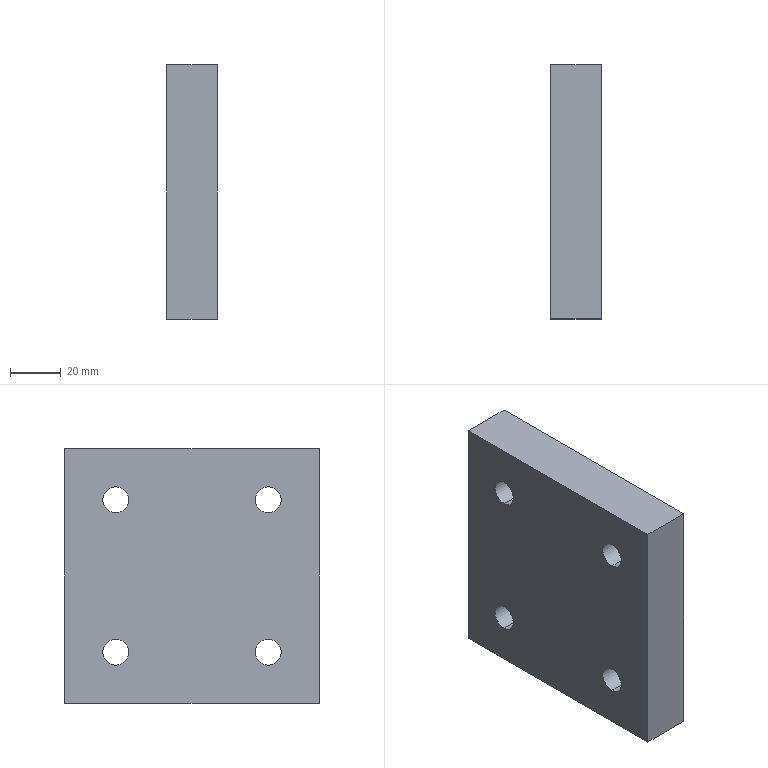Component | SolidWorks | THK-A1013Anti-CollisionBracketMountingPlate-1 | 1 solid | 14 faces | box 20 x 100 x 100 mm | volume 193463 mm3 | cylinder 8 | plane 6 | commonest cylinder face diameters 10.2 x8 | material Q235A
build123d program:
from build123d import *

# Parameters (mm, degrees)
SKETCH1_W           = 100
SKETCH1_H           = 100
BOSS_EXTRUDE1_DEPTH = 10
M12_TAPPED_HOLE1_D  = 10.2


with BuildPart() as part:
    # Sketch1 → Boss-Extrude1 (new, symmetric)
    with BuildSketch(Plane(origin=(0, 0, 0), x_dir=(0, 0, -1), z_dir=(1, 0, 0))):
        Rectangle(SKETCH1_W, SKETCH1_H)
    extrude(amount=BOSS_EXTRUDE1_DEPTH, both=True)

    # M12 Tapped Hole1 (through all)
    with Locations(Plane(origin=(10, 0, 0), x_dir=(0, 0, -1), z_dir=(1, 0, 0))):
        with Locations((-30, 30), (30, 30), (30, -30), (-30, -30)):
            Hole(M12_TAPPED_HOLE1_D / 2)


solid = part.part

# Placed as in the assembly
solid = solid.moved(Location((190, -105, -321), (0, 0, 0)))
STEP:
#1=COLOUR_RGB('',0.7922,0.8196,0.9333);
#2=FILL_AREA_STYLE_COLOUR('',#1);
#3=FILL_AREA_STYLE('',(#2));
#4=SURFACE_STYLE_FILL_AREA(#3);
#5=SURFACE_SIDE_STYLE('',(#4));
#6=SURFACE_STYLE_USAGE(.BOTH.,#5);
#7=PRESENTATION_STYLE_ASSIGNMENT((#6));
#8=CARTESIAN_POINT('',(7.087,-2.953,-11.256));
#9=VERTEX_POINT('',#8);
#10=CARTESIAN_POINT('',(7.087,-2.953,-11.657));
#11=VERTEX_POINT('',#10);
#12=CARTESIAN_POINT('',(7.087,-2.953,-11.457));
#13=DIRECTION('',(1.,0.,0.));
#14=DIRECTION('',(0.,0.,-1.));
#15=AXIS2_PLACEMENT_3D('',#12,#13,#14);
#16=CIRCLE('',#15,0.2008);
#17=EDGE_CURVE('',#9,#11,#16,.T.);
#18=ORIENTED_EDGE('',*,*,#17,.F.);
#19=CARTESIAN_POINT('',(7.874,-2.953,-11.256));
#20=VERTEX_POINT('',#19);
#21=CARTESIAN_POINT('',(7.874,-2.953,-11.256));
#22=DIRECTION('',(1.,0.,0.));
#23=VECTOR('',#22,39.37);
#24=LINE('',#21,#23);
#25=EDGE_CURVE('',#9,#20,#24,.T.);
#26=ORIENTED_EDGE('',*,*,#25,.T.);
#27=CARTESIAN_POINT('',(7.874,-2.953,-11.657));
#28=VERTEX_POINT('',#27);
#29=CARTESIAN_POINT('',(7.874,-2.953,-11.457));
#30=DIRECTION('',(1.,0.,0.));
#31=DIRECTION('',(0.,0.,-1.));
#32=AXIS2_PLACEMENT_3D('',#29,#30,#31);
#33=CIRCLE('',#32,0.2008);
#34=EDGE_CURVE('',#20,#28,#33,.T.);
#35=ORIENTED_EDGE('',*,*,#34,.T.);
#36=CARTESIAN_POINT('',(7.874,-2.953,-11.657));
#37=DIRECTION('',(1.,0.,0.));
#38=VECTOR('',#37,39.37);
#39=LINE('',#36,#38);
#40=EDGE_CURVE('',#11,#28,#39,.T.);
#41=ORIENTED_EDGE('',*,*,#40,.F.);
#42=EDGE_LOOP('',(#18,#26,#35,#41));
#43=FACE_OUTER_BOUND('',#42,.T.);
#44=CARTESIAN_POINT('',(7.874,-2.953,-11.457));
#45=DIRECTION('',(1.,0.,0.));
#46=DIRECTION('',(0.,0.,-1.));
#47=AXIS2_PLACEMENT_3D('',#44,#45,#46);
#48=CYLINDRICAL_SURFACE('',#47,0.2008);
#49=ADVANCED_FACE('',(#43),#48,.F.);
#50=CARTESIAN_POINT('',(7.087,-2.953,-13.618));
#51=VERTEX_POINT('',#50);
#52=CARTESIAN_POINT('',(7.087,-2.953,-14.02));
#53=VERTEX_POINT('',#52);
#54=CARTESIAN_POINT('',(7.087,-2.953,-13.819));
#55=DIRECTION('',(1.,0.,0.));
#56=DIRECTION('',(0.,0.,-1.));
#57=AXIS2_PLACEMENT_3D('',#54,#55,#56);
#58=CIRCLE('',#57,0.2008);
#59=EDGE_CURVE('',#51,#53,#58,.T.);
#60=ORIENTED_EDGE('',*,*,#59,.F.);
#61=CARTESIAN_POINT('',(7.874,-2.953,-13.618));
#62=VERTEX_POINT('',#61);
#63=CARTESIAN_POINT('',(7.874,-2.953,-13.618));
#64=DIRECTION('',(1.,0.,0.));
#65=VECTOR('',#64,39.37);
#66=LINE('',#63,#65);
#67=EDGE_CURVE('',#51,#62,#66,.T.);
#68=ORIENTED_EDGE('',*,*,#67,.T.);
#69=CARTESIAN_POINT('',(7.874,-2.953,-14.02));
#70=VERTEX_POINT('',#69);
#71=CARTESIAN_POINT('',(7.874,-2.953,-13.819));
#72=DIRECTION('',(1.,0.,0.));
#73=DIRECTION('',(0.,0.,-1.));
#74=AXIS2_PLACEMENT_3D('',#71,#72,#73);
#75=CIRCLE('',#74,0.2008);
#76=EDGE_CURVE('',#62,#70,#75,.T.);
#77=ORIENTED_EDGE('',*,*,#76,.T.);
#78=CARTESIAN_POINT('',(7.874,-2.953,-14.02));
#79=DIRECTION('',(1.,0.,0.));
#80=VECTOR('',#79,39.37);
#81=LINE('',#78,#80);
#82=EDGE_CURVE('',#53,#70,#81,.T.);
#83=ORIENTED_EDGE('',*,*,#82,.F.);
#84=EDGE_LOOP('',(#60,#68,#77,#83));
#85=FACE_OUTER_BOUND('',#84,.T.);
#86=CARTESIAN_POINT('',(7.874,-2.953,-13.819));
#87=DIRECTION('',(1.,0.,0.));
#88=DIRECTION('',(0.,0.,-1.));
#89=AXIS2_PLACEMENT_3D('',#86,#87,#88);
#90=CYLINDRICAL_SURFACE('',#89,0.2008);
#91=ADVANCED_FACE('',(#85),#90,.F.);
#92=CARTESIAN_POINT('',(7.087,-5.315,-13.618));
#93=VERTEX_POINT('',#92);
#94=CARTESIAN_POINT('',(7.087,-5.315,-14.02));
#95=VERTEX_POINT('',#94);
#96=CARTESIAN_POINT('',(7.087,-5.315,-13.819));
#97=DIRECTION('',(1.,0.,0.));
#98=DIRECTION('',(0.,0.,-1.));
#99=AXIS2_PLACEMENT_3D('',#96,#97,#98);
#100=CIRCLE('',#99,0.2008);
#101=EDGE_CURVE('',#93,#95,#100,.T.);
#102=ORIENTED_EDGE('',*,*,#101,.F.);
#103=CARTESIAN_POINT('',(7.874,-5.315,-13.618));
#104=VERTEX_POINT('',#103);
#105=CARTESIAN_POINT('',(7.874,-5.315,-13.618));
#106=DIRECTION('',(1.,0.,0.));
#107=VECTOR('',#106,39.37);
#108=LINE('',#105,#107);
#109=EDGE_CURVE('',#93,#104,#108,.T.);
#110=ORIENTED_EDGE('',*,*,#109,.T.);
#111=CARTESIAN_POINT('',(7.874,-5.315,-14.02));
#112=VERTEX_POINT('',#111);
#113=CARTESIAN_POINT('',(7.874,-5.315,-13.819));
#114=DIRECTION('',(1.,0.,0.));
#115=DIRECTION('',(0.,0.,-1.));
#116=AXIS2_PLACEMENT_3D('',#113,#114,#115);
#117=CIRCLE('',#116,0.2008);
#118=EDGE_CURVE('',#104,#112,#117,.T.);
#119=ORIENTED_EDGE('',*,*,#118,.T.);
#120=CARTESIAN_POINT('',(7.874,-5.315,-14.02));
#121=DIRECTION('',(1.,0.,0.));
#122=VECTOR('',#121,39.37);
#123=LINE('',#120,#122);
#124=EDGE_CURVE('',#95,#112,#123,.T.);
#125=ORIENTED_EDGE('',*,*,#124,.F.);
#126=EDGE_LOOP('',(#102,#110,#119,#125));
#127=FACE_OUTER_BOUND('',#126,.T.);
#128=CARTESIAN_POINT('',(7.874,-5.315,-13.819));
#129=DIRECTION('',(1.,0.,0.));
#130=DIRECTION('',(0.,0.,-1.));
#131=AXIS2_PLACEMENT_3D('',#128,#129,#130);
#132=CYLINDRICAL_SURFACE('',#131,0.2008);
#133=ADVANCED_FACE('',(#127),#132,.F.);
#134=CARTESIAN_POINT('',(7.087,-5.315,-11.256));
#135=VERTEX_POINT('',#134);
#136=CARTESIAN_POINT('',(7.087,-5.315,-11.657));
#137=VERTEX_POINT('',#136);
#138=CARTESIAN_POINT('',(7.087,-5.315,-11.457));
#139=DIRECTION('',(1.,0.,0.));
#140=DIRECTION('',(0.,0.,-1.));
#141=AXIS2_PLACEMENT_3D('',#138,#139,#140);
#142=CIRCLE('',#141,0.2008);
#143=EDGE_CURVE('',#135,#137,#142,.T.);
#144=ORIENTED_EDGE('',*,*,#143,.F.);
#145=CARTESIAN_POINT('',(7.874,-5.315,-11.256));
#146=VERTEX_POINT('',#145);
#147=CARTESIAN_POINT('',(7.874,-5.315,-11.256));
#148=DIRECTION('',(1.,0.,0.));
#149=VECTOR('',#148,39.37);
#150=LINE('',#147,#149);
#151=EDGE_CURVE('',#135,#146,#150,.T.);
#152=ORIENTED_EDGE('',*,*,#151,.T.);
#153=CARTESIAN_POINT('',(7.874,-5.315,-11.657));
#154=VERTEX_POINT('',#153);
#155=CARTESIAN_POINT('',(7.874,-5.315,-11.457));
#156=DIRECTION('',(1.,0.,0.));
#157=DIRECTION('',(0.,0.,-1.));
#158=AXIS2_PLACEMENT_3D('',#155,#156,#157);
#159=CIRCLE('',#158,0.2008);
#160=EDGE_CURVE('',#146,#154,#159,.T.);
#161=ORIENTED_EDGE('',*,*,#160,.T.);
#162=CARTESIAN_POINT('',(7.874,-5.315,-11.657));
#163=DIRECTION('',(1.,0.,0.));
#164=VECTOR('',#163,39.37);
#165=LINE('',#162,#164);
#166=EDGE_CURVE('',#137,#154,#165,.T.);
#167=ORIENTED_EDGE('',*,*,#166,.F.);
#168=EDGE_LOOP('',(#144,#152,#161,#167));
#169=FACE_OUTER_BOUND('',#168,.T.);
#170=CARTESIAN_POINT('',(7.874,-5.315,-11.457));
#171=DIRECTION('',(1.,0.,0.));
#172=DIRECTION('',(0.,0.,-1.));
#173=AXIS2_PLACEMENT_3D('',#170,#171,#172);
#174=CYLINDRICAL_SURFACE('',#173,0.2008);
#175=ADVANCED_FACE('',(#169),#174,.F.);
#176=CARTESIAN_POINT('',(7.087,-6.102,-14.606));
#177=VERTEX_POINT('',#176);
#178=CARTESIAN_POINT('',(7.087,-2.165,-14.606));
#179=VERTEX_POINT('',#178);
#180=CARTESIAN_POINT('',(7.087,-6.102,-14.606));
#181=DIRECTION('',(0.,1.,0.));
#182=VECTOR('',#181,39.37);
#183=LINE('',#180,#182);
#184=EDGE_CURVE('',#177,#179,#183,.T.);
#185=ORIENTED_EDGE('',*,*,#184,.T.);
#186=CARTESIAN_POINT('',(7.874,-2.165,-14.606));
#187=VERTEX_POINT('',#186);
#188=CARTESIAN_POINT('',(7.874,-2.165,-14.606));
#189=DIRECTION('',(-1.,0.,0.));
#190=VECTOR('',#189,39.37);
#191=LINE('',#188,#190);
#192=EDGE_CURVE('',#187,#179,#191,.T.);
#193=ORIENTED_EDGE('',*,*,#192,.F.);
#194=CARTESIAN_POINT('',(7.874,-6.102,-14.606));
#195=VERTEX_POINT('',#194);
#196=CARTESIAN_POINT('',(7.874,-6.102,-14.606));
#197=DIRECTION('',(0.,1.,0.));
#198=VECTOR('',#197,39.37);
#199=LINE('',#196,#198);
#200=EDGE_CURVE('',#195,#187,#199,.T.);
#201=ORIENTED_EDGE('',*,*,#200,.F.);
#202=CARTESIAN_POINT('',(7.874,-6.102,-14.606));
#203=DIRECTION('',(-1.,0.,0.));
#204=VECTOR('',#203,39.37);
#205=LINE('',#202,#204);
#206=EDGE_CURVE('',#195,#177,#205,.T.);
#207=ORIENTED_EDGE('',*,*,#206,.T.);
#208=EDGE_LOOP('',(#185,#193,#201,#207));
#209=FACE_OUTER_BOUND('',#208,.T.);
#210=CARTESIAN_POINT('',(7.874,-6.102,-14.606));
#211=DIRECTION('',(0.,0.,1.));
#212=DIRECTION('',(1.,0.,0.));
#213=AXIS2_PLACEMENT_3D('',#210,#211,#212);
#214=PLANE('',#213);
#215=ADVANCED_FACE('',(#209),#214,.F.);
#216=CARTESIAN_POINT('',(7.087,-2.165,-10.669));
#217=VERTEX_POINT('',#216);
#218=CARTESIAN_POINT('',(7.087,-2.165,-10.669));
#219=DIRECTION('',(0.,0.,1.));
#220=VECTOR('',#219,39.37);
#221=LINE('',#218,#220);
#222=EDGE_CURVE('',#179,#217,#221,.T.);
#223=ORIENTED_EDGE('',*,*,#222,.T.);
#224=CARTESIAN_POINT('',(7.874,-2.165,-10.669));
#225=VERTEX_POINT('',#224);
#226=CARTESIAN_POINT('',(7.874,-2.165,-10.669));
#227=DIRECTION('',(-1.,0.,0.));
#228=VECTOR('',#227,39.37);
#229=LINE('',#226,#228);
#230=EDGE_CURVE('',#225,#217,#229,.T.);
#231=ORIENTED_EDGE('',*,*,#230,.F.);
#232=CARTESIAN_POINT('',(7.874,-2.165,-10.669));
#233=DIRECTION('',(0.,0.,1.));
#234=VECTOR('',#233,39.37);
#235=LINE('',#232,#234);
#236=EDGE_CURVE('',#187,#225,#235,.T.);
#237=ORIENTED_EDGE('',*,*,#236,.F.);
#238=ORIENTED_EDGE('',*,*,#192,.T.);
#239=EDGE_LOOP('',(#223,#231,#237,#238));
#240=FACE_OUTER_BOUND('',#239,.T.);
#241=CARTESIAN_POINT('',(7.874,-2.165,-10.669));
#242=DIRECTION('',(0.,-1.,0.));
#243=DIRECTION('',(0.,0.,-1.));
#244=AXIS2_PLACEMENT_3D('',#241,#242,#243);
#245=PLANE('',#244);
#246=ADVANCED_FACE('',(#240),#245,.F.);
#247=CARTESIAN_POINT('',(7.087,-6.102,-10.669));
#248=VERTEX_POINT('',#247);
#249=CARTESIAN_POINT('',(7.087,-6.102,-10.669));
#250=DIRECTION('',(0.,-1.,0.));
#251=VECTOR('',#250,39.37);
#252=LINE('',#249,#251);
#253=EDGE_CURVE('',#217,#248,#252,.T.);
#254=ORIENTED_EDGE('',*,*,#253,.T.);
#255=CARTESIAN_POINT('',(7.874,-6.102,-10.669));
#256=VERTEX_POINT('',#255);
#257=CARTESIAN_POINT('',(7.874,-6.102,-10.669));
#258=DIRECTION('',(-1.,0.,0.));
#259=VECTOR('',#258,39.37);
#260=LINE('',#257,#259);
#261=EDGE_CURVE('',#256,#248,#260,.T.);
#262=ORIENTED_EDGE('',*,*,#261,.F.);
#263=CARTESIAN_POINT('',(7.874,-6.102,-10.669));
#264=DIRECTION('',(0.,-1.,0.));
#265=VECTOR('',#264,39.37);
#266=LINE('',#263,#265);
#267=EDGE_CURVE('',#225,#256,#266,.T.);
#268=ORIENTED_EDGE('',*,*,#267,.F.);
#269=ORIENTED_EDGE('',*,*,#230,.T.);
#270=EDGE_LOOP('',(#254,#262,#268,#269));
#271=FACE_OUTER_BOUND('',#270,.T.);
#272=CARTESIAN_POINT('',(7.874,-6.102,-10.669));
#273=DIRECTION('',(0.,0.,-1.));
#274=DIRECTION('',(-1.,0.,0.));
#275=AXIS2_PLACEMENT_3D('',#272,#273,#274);
#276=PLANE('',#275);
#277=ADVANCED_FACE('',(#271),#276,.F.);
#278=CARTESIAN_POINT('',(7.087,-6.102,-10.669));
#279=DIRECTION('',(0.,0.,-1.));
#280=VECTOR('',#279,39.37);
#281=LINE('',#278,#280);
#282=EDGE_CURVE('',#248,#177,#281,.T.);
#283=ORIENTED_EDGE('',*,*,#282,.T.);
#284=ORIENTED_EDGE('',*,*,#206,.F.);
#285=CARTESIAN_POINT('',(7.874,-6.102,-10.669));
#286=DIRECTION('',(0.,0.,-1.));
#287=VECTOR('',#286,39.37);
#288=LINE('',#285,#287);
#289=EDGE_CURVE('',#256,#195,#288,.T.);
#290=ORIENTED_EDGE('',*,*,#289,.F.);
#291=ORIENTED_EDGE('',*,*,#261,.T.);
#292=EDGE_LOOP('',(#283,#284,#290,#291));
#293=FACE_OUTER_BOUND('',#292,.T.);
#294=CARTESIAN_POINT('',(7.874,-6.102,-10.669));
#295=DIRECTION('',(0.,1.,0.));
#296=DIRECTION('',(0.,0.,1.));
#297=AXIS2_PLACEMENT_3D('',#294,#295,#296);
#298=PLANE('',#297);
#299=ADVANCED_FACE('',(#293),#298,.F.);
#300=CARTESIAN_POINT('',(7.874,-2.953,-11.457));
#301=DIRECTION('',(1.,0.,0.));
#302=DIRECTION('',(0.,0.,-1.));
#303=AXIS2_PLACEMENT_3D('',#300,#301,#302);
#304=CIRCLE('',#303,0.2008);
#305=EDGE_CURVE('',#28,#20,#304,.T.);
#306=ORIENTED_EDGE('',*,*,#305,.F.);
#307=ORIENTED_EDGE('',*,*,#34,.F.);
#308=EDGE_LOOP('',(#306,#307));
#309=FACE_BOUND('',#308,.T.);
#310=CARTESIAN_POINT('',(7.874,-2.953,-13.819));
#311=DIRECTION('',(1.,0.,0.));
#312=DIRECTION('',(0.,0.,-1.));
#313=AXIS2_PLACEMENT_3D('',#310,#311,#312);
#314=CIRCLE('',#313,0.2008);
#315=EDGE_CURVE('',#70,#62,#314,.T.);
#316=ORIENTED_EDGE('',*,*,#315,.F.);
#317=ORIENTED_EDGE('',*,*,#76,.F.);
#318=EDGE_LOOP('',(#316,#317));
#319=FACE_BOUND('',#318,.T.);
#320=CARTESIAN_POINT('',(7.874,-5.315,-13.819));
#321=DIRECTION('',(1.,0.,0.));
#322=DIRECTION('',(0.,0.,-1.));
#323=AXIS2_PLACEMENT_3D('',#320,#321,#322);
#324=CIRCLE('',#323,0.2008);
#325=EDGE_CURVE('',#112,#104,#324,.T.);
#326=ORIENTED_EDGE('',*,*,#325,.F.);
#327=ORIENTED_EDGE('',*,*,#118,.F.);
#328=EDGE_LOOP('',(#326,#327));
#329=FACE_BOUND('',#328,.T.);
#330=CARTESIAN_POINT('',(7.874,-5.315,-11.457));
#331=DIRECTION('',(1.,0.,0.));
#332=DIRECTION('',(0.,0.,-1.));
#333=AXIS2_PLACEMENT_3D('',#330,#331,#332);
#334=CIRCLE('',#333,0.2008);
#335=EDGE_CURVE('',#154,#146,#334,.T.);
#336=ORIENTED_EDGE('',*,*,#335,.F.);
#337=ORIENTED_EDGE('',*,*,#160,.F.);
#338=EDGE_LOOP('',(#336,#337));
#339=FACE_BOUND('',#338,.T.);
#340=ORIENTED_EDGE('',*,*,#200,.T.);
#341=ORIENTED_EDGE('',*,*,#236,.T.);
#342=ORIENTED_EDGE('',*,*,#267,.T.);
#343=ORIENTED_EDGE('',*,*,#289,.T.);
#344=EDGE_LOOP('',(#340,#341,#342,#343));
#345=FACE_OUTER_BOUND('',#344,.T.);
#346=CARTESIAN_POINT('',(7.874,-4.134,-12.638));
#347=DIRECTION('',(-1.,0.,0.));
#348=DIRECTION('',(0.,0.,1.));
#349=AXIS2_PLACEMENT_3D('',#346,#347,#348);
#350=PLANE('',#349);
#351=ADVANCED_FACE('',(#309,#319,#329,#339,#345),#350,.F.);
#352=CARTESIAN_POINT('',(7.087,-2.953,-11.457));
#353=DIRECTION('',(1.,0.,0.));
#354=DIRECTION('',(0.,0.,-1.));
#355=AXIS2_PLACEMENT_3D('',#352,#353,#354);
#356=CIRCLE('',#355,0.2008);
#357=EDGE_CURVE('',#11,#9,#356,.T.);
#358=ORIENTED_EDGE('',*,*,#357,.T.);
#359=ORIENTED_EDGE('',*,*,#17,.T.);
#360=EDGE_LOOP('',(#358,#359));
#361=FACE_BOUND('',#360,.T.);
#362=CARTESIAN_POINT('',(7.087,-2.953,-13.819));
#363=DIRECTION('',(1.,0.,0.));
#364=DIRECTION('',(0.,0.,-1.));
#365=AXIS2_PLACEMENT_3D('',#362,#363,#364);
#366=CIRCLE('',#365,0.2008);
#367=EDGE_CURVE('',#53,#51,#366,.T.);
#368=ORIENTED_EDGE('',*,*,#367,.T.);
#369=ORIENTED_EDGE('',*,*,#59,.T.);
#370=EDGE_LOOP('',(#368,#369));
#371=FACE_BOUND('',#370,.T.);
#372=CARTESIAN_POINT('',(7.087,-5.315,-13.819));
#373=DIRECTION('',(1.,0.,0.));
#374=DIRECTION('',(0.,0.,-1.));
#375=AXIS2_PLACEMENT_3D('',#372,#373,#374);
#376=CIRCLE('',#375,0.2008);
#377=EDGE_CURVE('',#95,#93,#376,.T.);
#378=ORIENTED_EDGE('',*,*,#377,.T.);
#379=ORIENTED_EDGE('',*,*,#101,.T.);
#380=EDGE_LOOP('',(#378,#379));
#381=FACE_BOUND('',#380,.T.);
#382=CARTESIAN_POINT('',(7.087,-5.315,-11.457));
#383=DIRECTION('',(1.,0.,0.));
#384=DIRECTION('',(0.,0.,-1.));
#385=AXIS2_PLACEMENT_3D('',#382,#383,#384);
#386=CIRCLE('',#385,0.2008);
#387=EDGE_CURVE('',#137,#135,#386,.T.);
#388=ORIENTED_EDGE('',*,*,#387,.T.);
#389=ORIENTED_EDGE('',*,*,#143,.T.);
#390=EDGE_LOOP('',(#388,#389));
#391=FACE_BOUND('',#390,.T.);
#392=ORIENTED_EDGE('',*,*,#184,.F.);
#393=ORIENTED_EDGE('',*,*,#282,.F.);
#394=ORIENTED_EDGE('',*,*,#253,.F.);
#395=ORIENTED_EDGE('',*,*,#222,.F.);
#396=EDGE_LOOP('',(#392,#393,#394,#395));
#397=FACE_OUTER_BOUND('',#396,.T.);
#398=CARTESIAN_POINT('',(7.087,-4.134,-12.638));
#399=DIRECTION('',(-1.,0.,0.));
#400=DIRECTION('',(0.,0.,1.));
#401=AXIS2_PLACEMENT_3D('',#398,#399,#400);
#402=PLANE('',#401);
#403=ADVANCED_FACE('',(#361,#371,#381,#391,#397),#402,.T.);
#404=ORIENTED_EDGE('',*,*,#151,.F.);
#405=ORIENTED_EDGE('',*,*,#387,.F.);
#406=ORIENTED_EDGE('',*,*,#166,.T.);
#407=ORIENTED_EDGE('',*,*,#335,.T.);
#408=EDGE_LOOP('',(#404,#405,#406,#407));
#409=FACE_OUTER_BOUND('',#408,.T.);
#410=CARTESIAN_POINT('',(7.874,-5.315,-11.457));
#411=DIRECTION('',(1.,0.,0.));
#412=DIRECTION('',(0.,0.,-1.));
#413=AXIS2_PLACEMENT_3D('',#410,#411,#412);
#414=CYLINDRICAL_SURFACE('',#413,0.2008);
#415=ADVANCED_FACE('',(#409),#414,.F.);
#416=ORIENTED_EDGE('',*,*,#109,.F.);
#417=ORIENTED_EDGE('',*,*,#377,.F.);
#418=ORIENTED_EDGE('',*,*,#124,.T.);
#419=ORIENTED_EDGE('',*,*,#325,.T.);
#420=EDGE_LOOP('',(#416,#417,#418,#419));
#421=FACE_OUTER_BOUND('',#420,.T.);
#422=CARTESIAN_POINT('',(7.874,-5.315,-13.819));
#423=DIRECTION('',(1.,0.,0.));
#424=DIRECTION('',(0.,0.,-1.));
#425=AXIS2_PLACEMENT_3D('',#422,#423,#424);
#426=CYLINDRICAL_SURFACE('',#425,0.2008);
#427=ADVANCED_FACE('',(#421),#426,.F.);
#428=ORIENTED_EDGE('',*,*,#67,.F.);
#429=ORIENTED_EDGE('',*,*,#367,.F.);
#430=ORIENTED_EDGE('',*,*,#82,.T.);
#431=ORIENTED_EDGE('',*,*,#315,.T.);
#432=EDGE_LOOP('',(#428,#429,#430,#431));
#433=FACE_OUTER_BOUND('',#432,.T.);
#434=CARTESIAN_POINT('',(7.874,-2.953,-13.819));
#435=DIRECTION('',(1.,0.,0.));
#436=DIRECTION('',(0.,0.,-1.));
#437=AXIS2_PLACEMENT_3D('',#434,#435,#436);
#438=CYLINDRICAL_SURFACE('',#437,0.2008);
#439=ADVANCED_FACE('',(#433),#438,.F.);
#440=ORIENTED_EDGE('',*,*,#25,.F.);
#441=ORIENTED_EDGE('',*,*,#357,.F.);
#442=ORIENTED_EDGE('',*,*,#40,.T.);
#443=ORIENTED_EDGE('',*,*,#305,.T.);
#444=EDGE_LOOP('',(#440,#441,#442,#443));
#445=FACE_OUTER_BOUND('',#444,.T.);
#446=CARTESIAN_POINT('',(7.874,-2.953,-11.457));
#447=DIRECTION('',(1.,0.,0.));
#448=DIRECTION('',(0.,0.,-1.));
#449=AXIS2_PLACEMENT_3D('',#446,#447,#448);
#450=CYLINDRICAL_SURFACE('',#449,0.2008);
#451=ADVANCED_FACE('',(#445),#450,.F.);
#452=CLOSED_SHELL('',(#49,#91,#133,#175,#215,#246,#277,#299,#351,#403,#415,#427,#439,#451));
#453=MANIFOLD_SOLID_BREP('',#452);
#454=STYLED_ITEM('',(#7),#453);
#455=PRESENTATION_LAYER_ASSIGNMENT('','',(#454));
#456=(LENGTH_UNIT()NAMED_UNIT(*)SI_UNIT($,.METRE.));
#457=LENGTH_MEASURE_WITH_UNIT(LENGTH_MEASURE(0.0254),#456);
#458=DIMENSIONAL_EXPONENTS(1.,0.,0.,0.,0.,0.,0.);
#459=(CONVERSION_BASED_UNIT('',#457)LENGTH_UNIT()NAMED_UNIT(#458));
#460=UNCERTAINTY_MEASURE_WITH_UNIT(LENGTH_MEASURE(0.00001),#459,'','');
#461=(NAMED_UNIT(*)PLANE_ANGLE_UNIT()SI_UNIT($,.RADIAN.));
#462=(NAMED_UNIT(*)SI_UNIT($,.STERADIAN.)SOLID_ANGLE_UNIT());
#463=(GEOMETRIC_REPRESENTATION_CONTEXT(3)GLOBAL_UNCERTAINTY_ASSIGNED_CONTEXT((#460))GLOBAL_UNIT_ASSIGNED_CONTEXT((#459,#461,#462))REPRESENTATION_CONTEXT('',''));
#464=MECHANICAL_DESIGN_GEOMETRIC_PRESENTATION_REPRESENTATION('',(#454),#463);
#465=CARTESIAN_POINT('',(0.,0.,0.));
#466=DIRECTION('',(0.,0.,1.));
#467=DIRECTION('',(1.,0.,0.));
#468=AXIS2_PLACEMENT_3D('',#465,#466,#467);
#469=(LENGTH_UNIT()NAMED_UNIT(*)SI_UNIT($,.METRE.));
#470=LENGTH_MEASURE_WITH_UNIT(LENGTH_MEASURE(0.0254),#469);
#471=DIMENSIONAL_EXPONENTS(1.,0.,0.,0.,0.,0.,0.);
#472=(CONVERSION_BASED_UNIT('',#470)LENGTH_UNIT()NAMED_UNIT(#471));
#473=UNCERTAINTY_MEASURE_WITH_UNIT(LENGTH_MEASURE(0.00001),#472,'','');
#474=(NAMED_UNIT(*)PLANE_ANGLE_UNIT()SI_UNIT($,.RADIAN.));
#475=(NAMED_UNIT(*)SI_UNIT($,.STERADIAN.)SOLID_ANGLE_UNIT());
#476=(GEOMETRIC_REPRESENTATION_CONTEXT(3)GLOBAL_UNCERTAINTY_ASSIGNED_CONTEXT((#473))GLOBAL_UNIT_ASSIGNED_CONTEXT((#472,#474,#475))REPRESENTATION_CONTEXT('',''));
#477=ADVANCED_BREP_SHAPE_REPRESENTATION('',(#453,#468),#476);